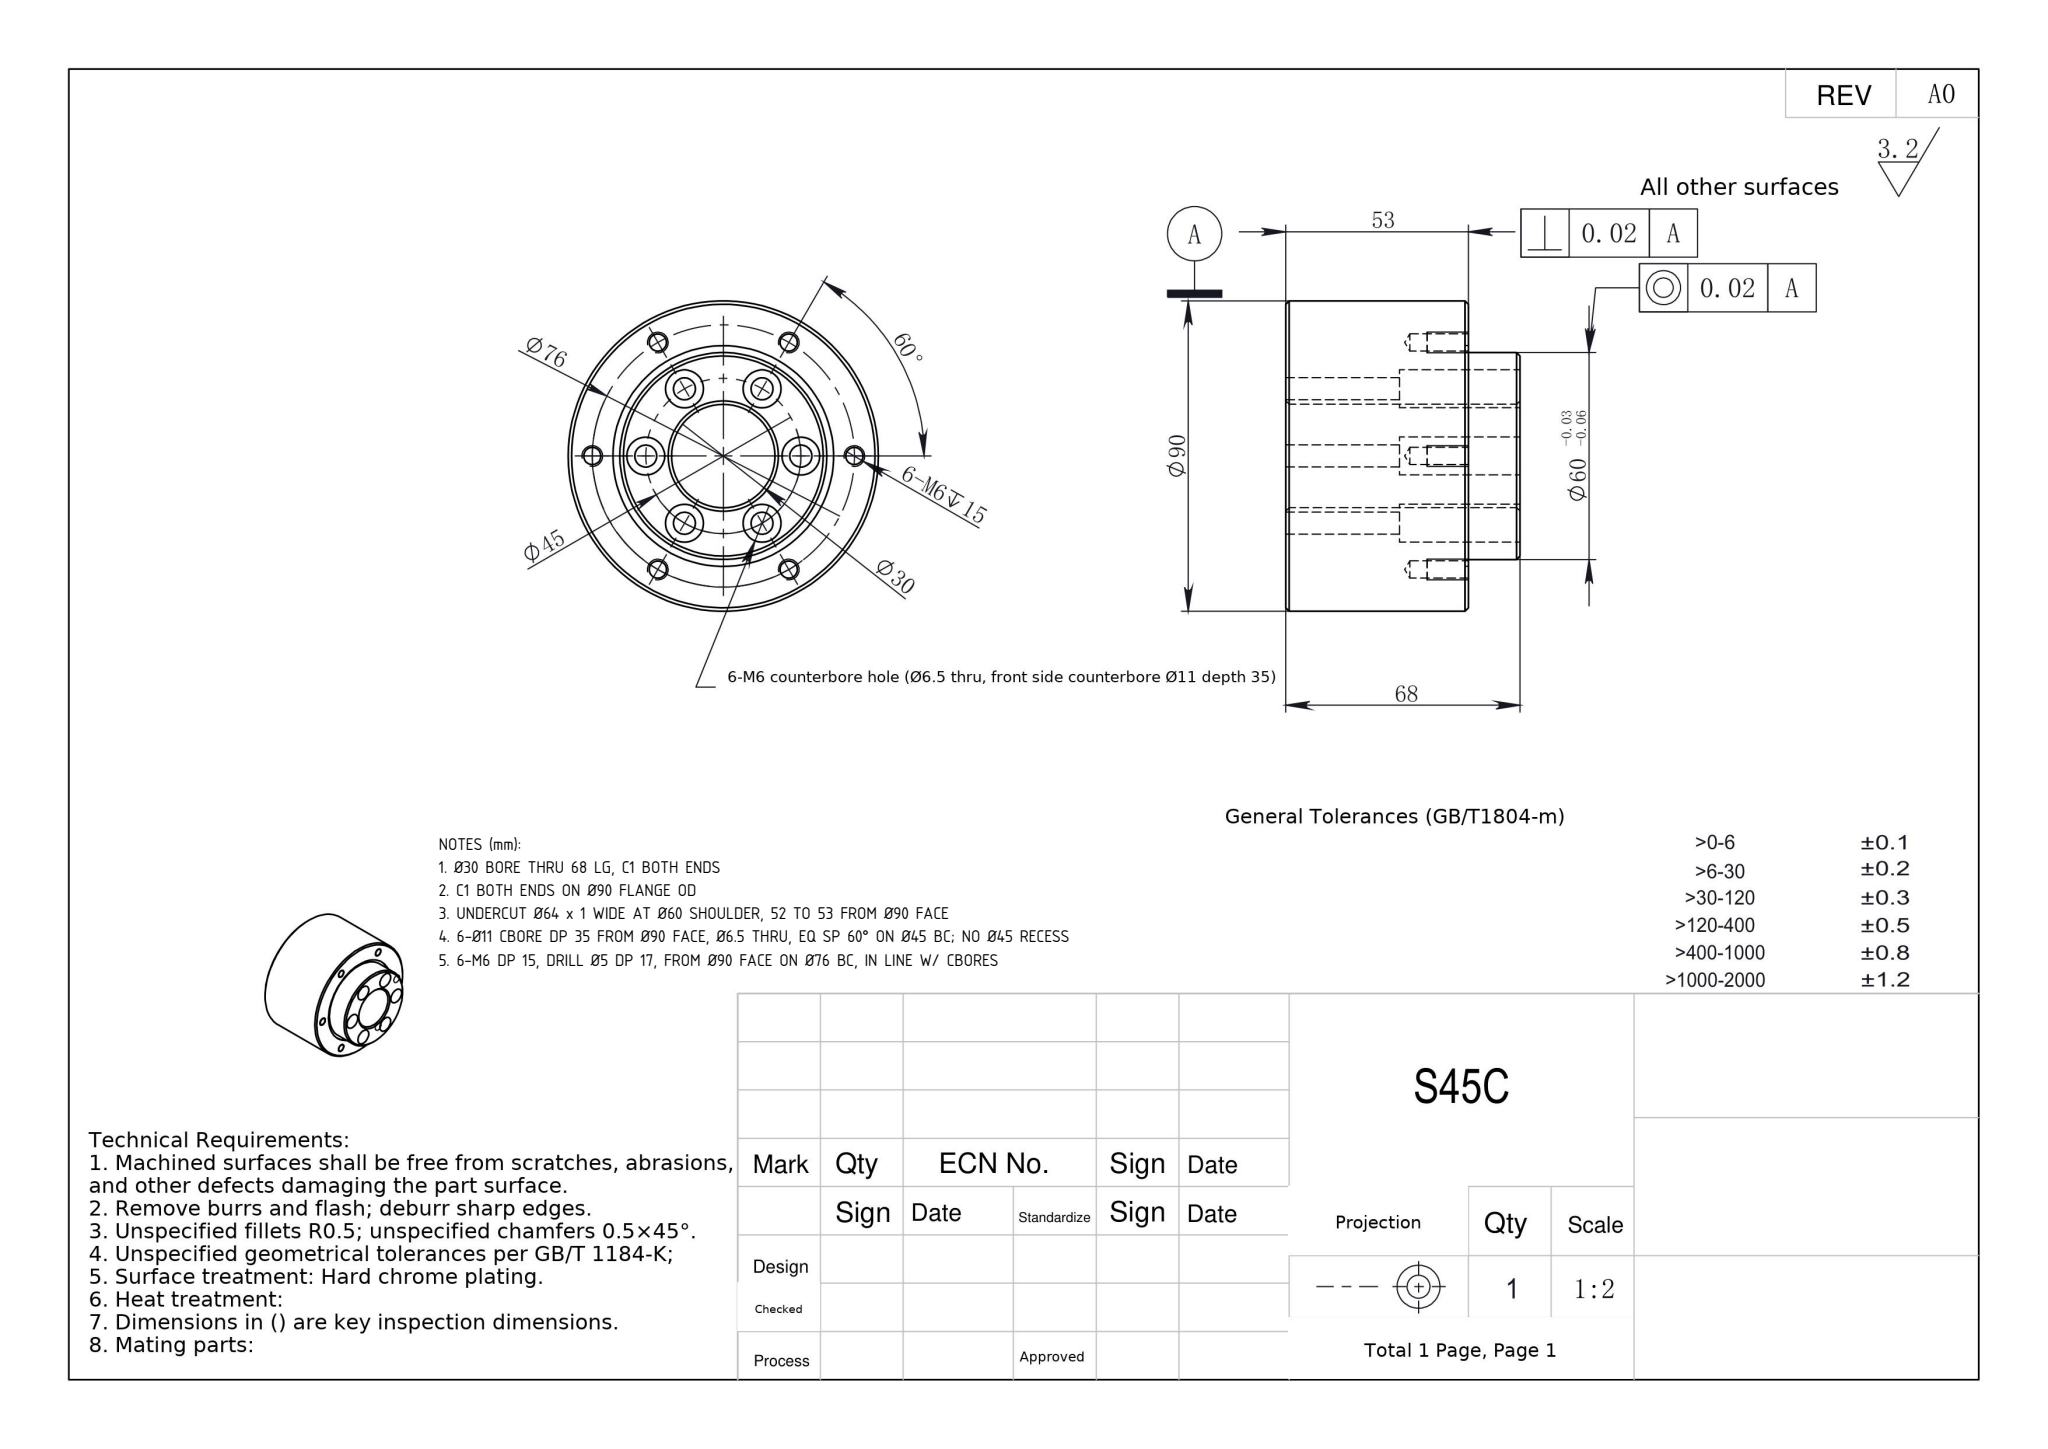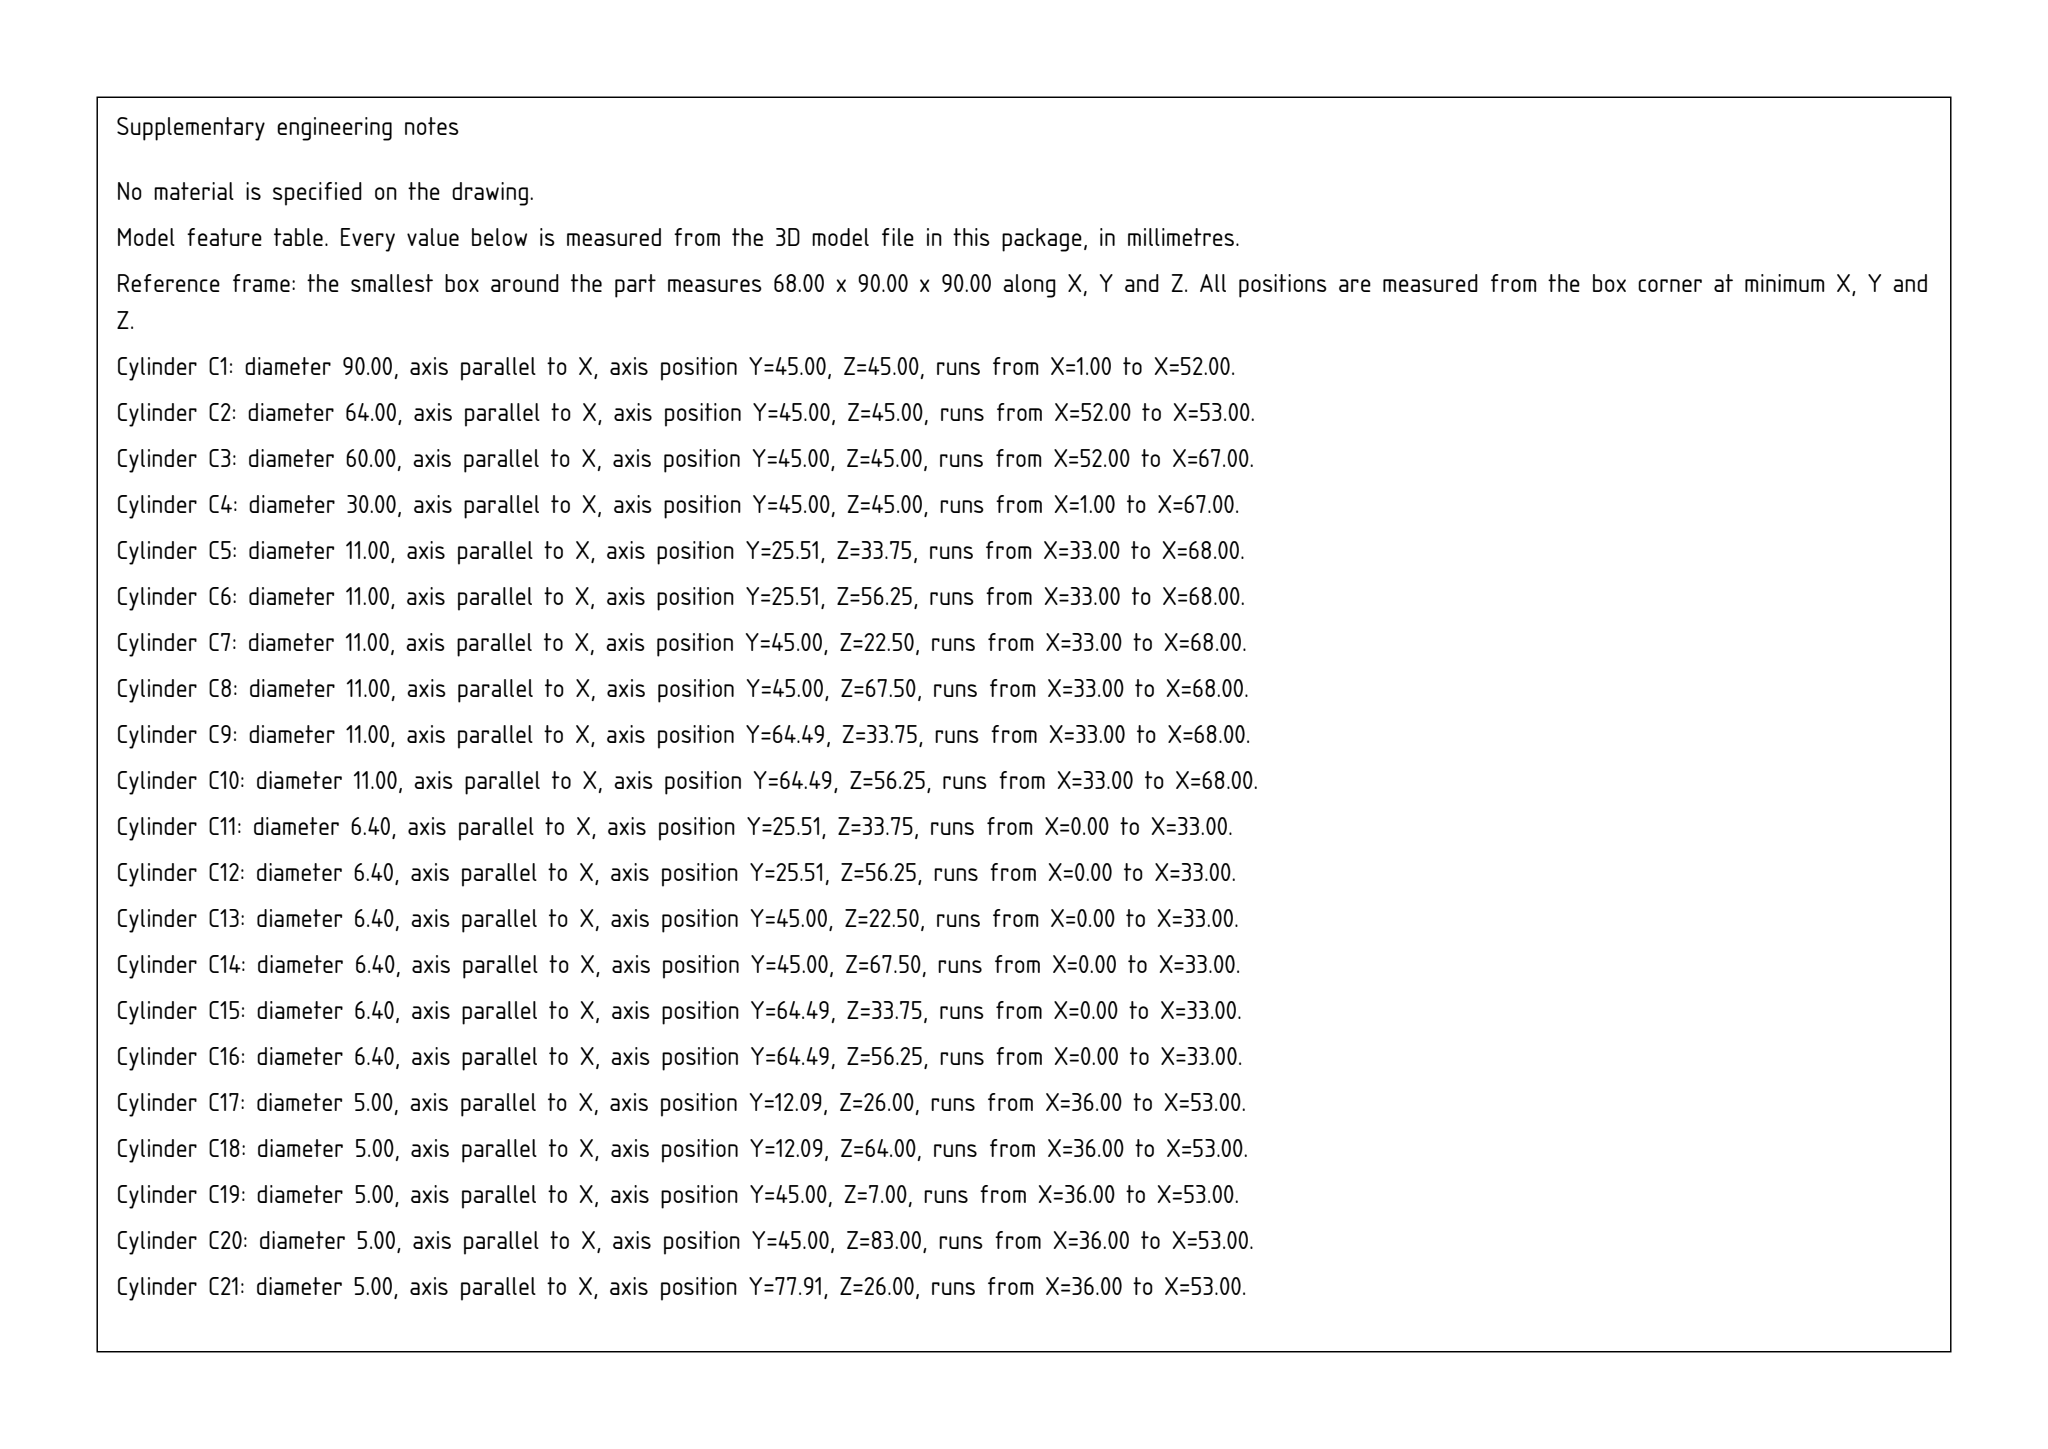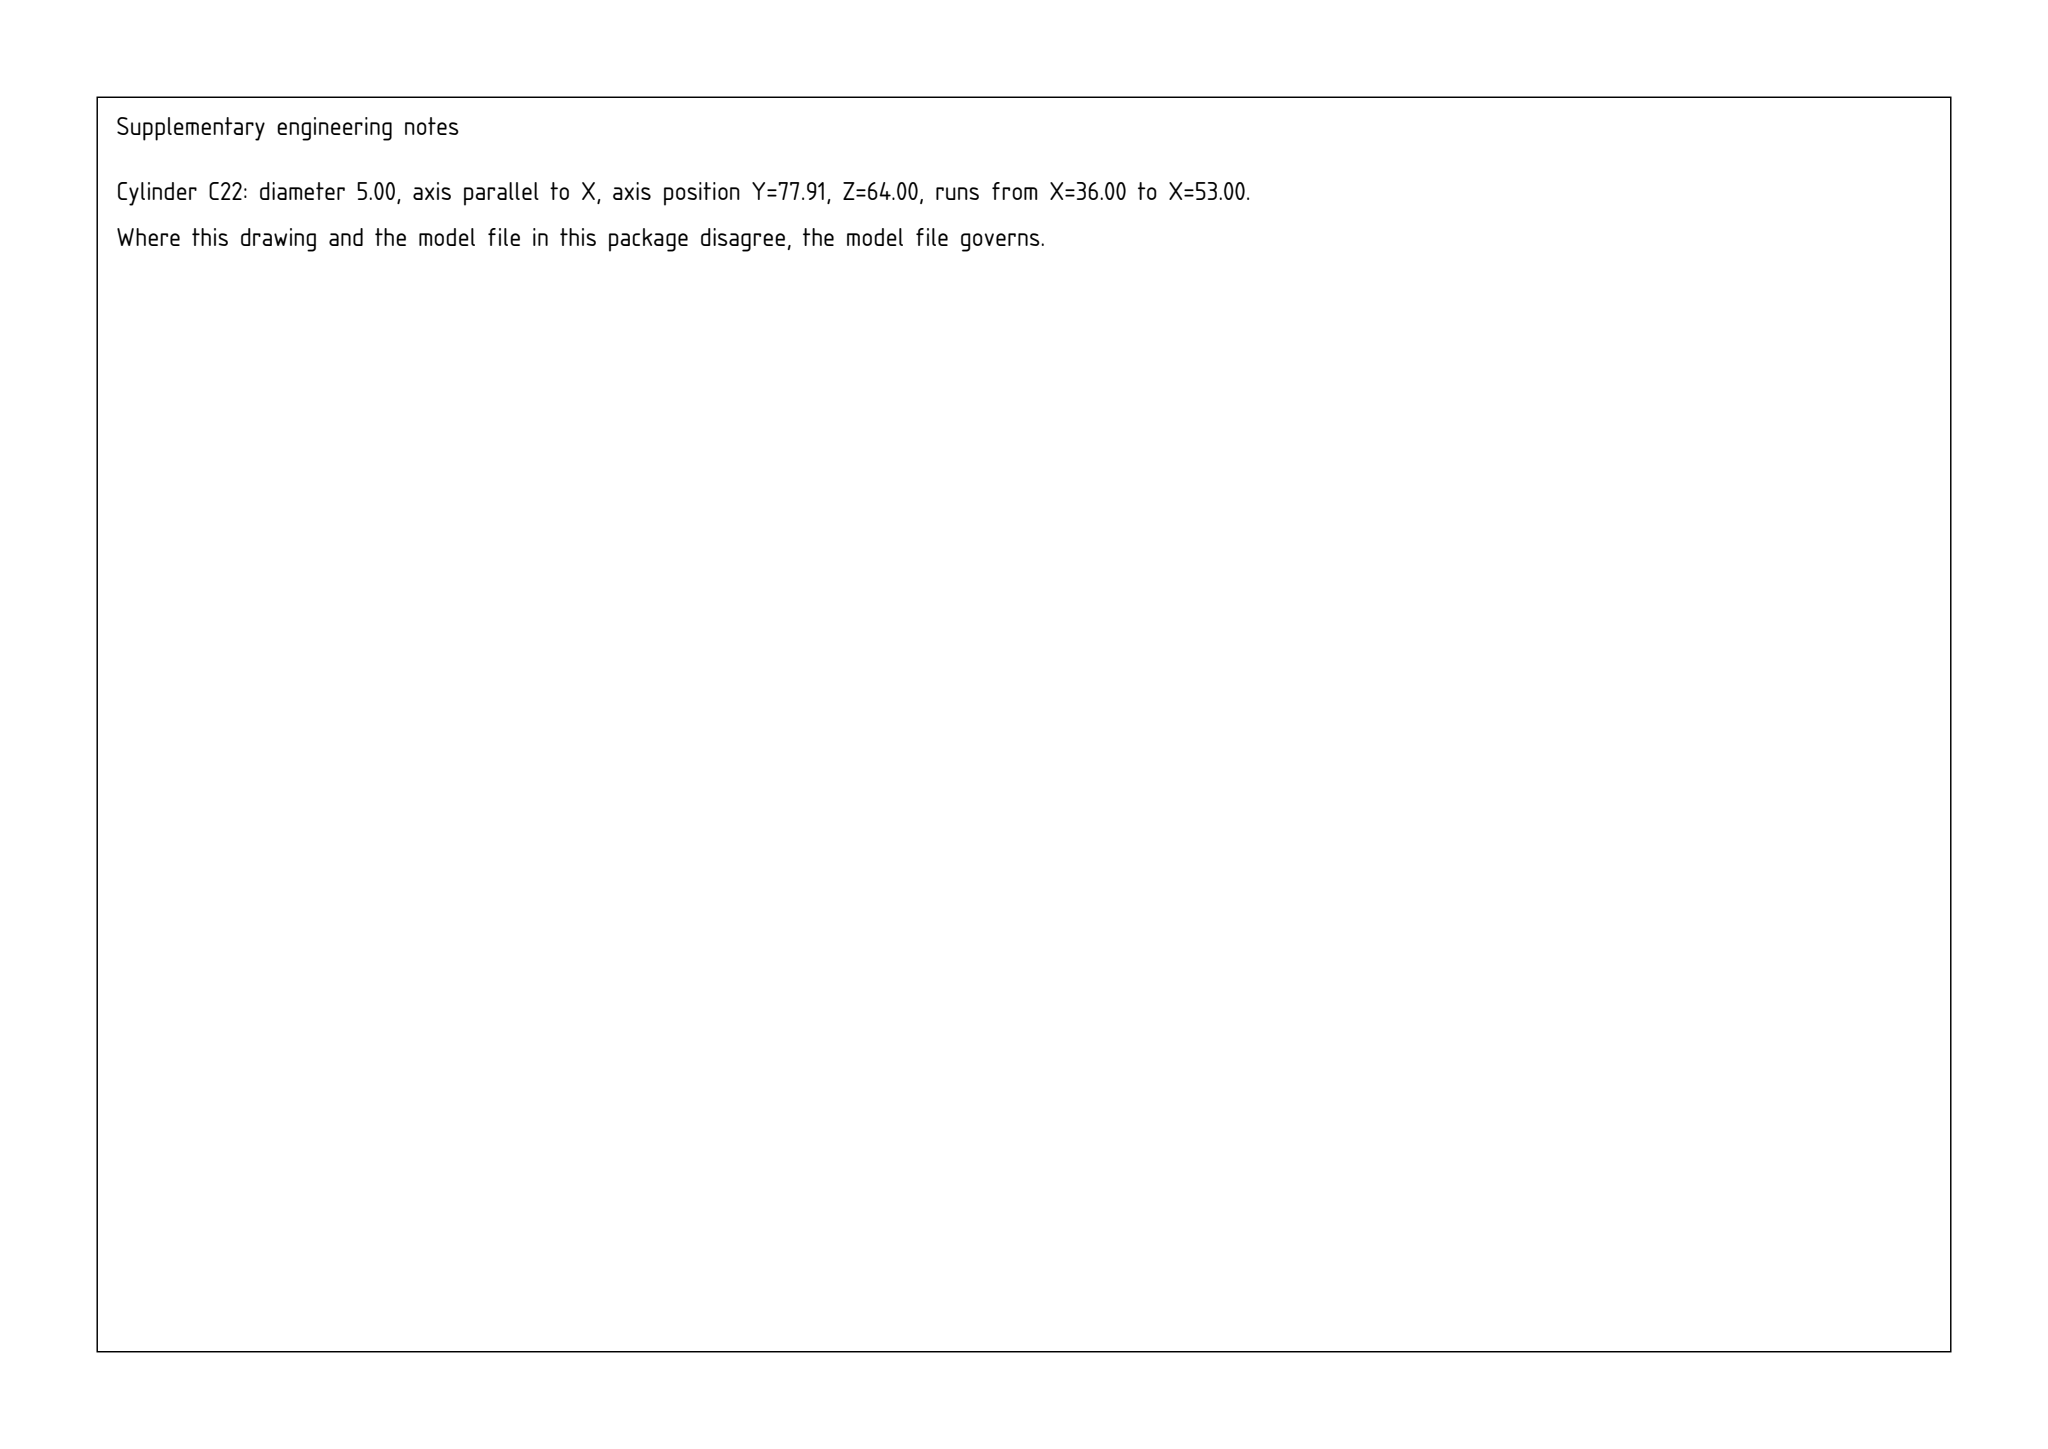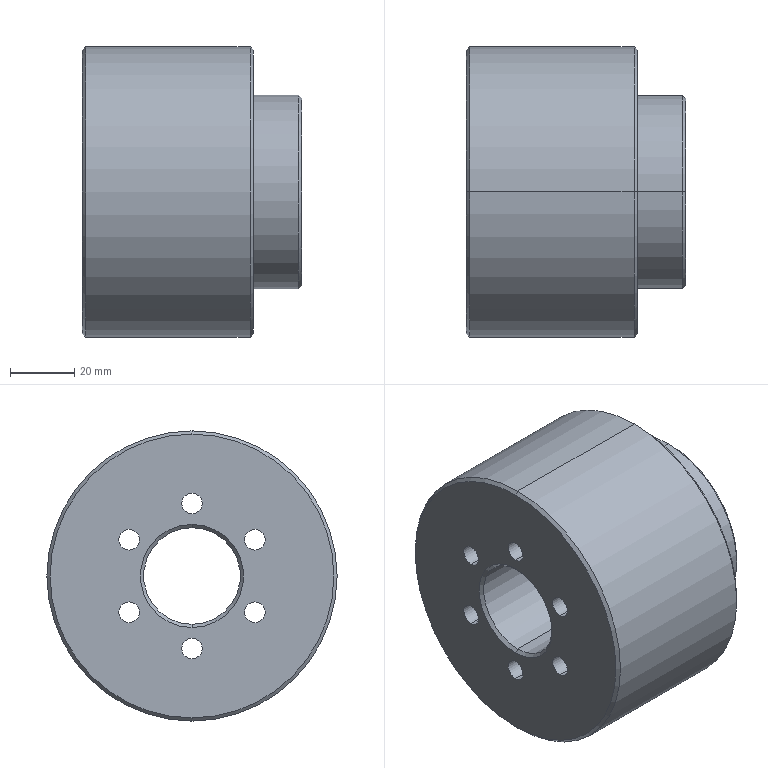Part | SolidWorks | mm | 1 solid | 76 faces | box 68 x 90 x 90 mm | volume 302268 mm3 | cylinder 44 | cone 22 | plane 10 | commonest cylinder face diameters 11 x12 6.4 x12 5 x12 60 x2 64 x2 90 x2 30 x2
Drawing notes:
Ø30 BORE THRU 68 LG, C1 BOTH ENDS | from the solid: Ø30 cyl L=66 on x axis + 90° cones ref Ø30/Ø32 each end = 68 total = bbox X
C1 BOTH ENDS ON Ø90 FLANGE OD | from the solid: 90° cones ref dia 90 and 88 at x=0-1 and x=52-53 => 1x45°
UNDERCUT Ø64 x 1 WIDE AT Ø60 SHOULDER, 52 TO 53 FROM Ø90 FACE | from the solid: Cyl Ø64 axis x L=1 spanning x=52 to 53; shoulder plane at x=53
6-Ø11 CBORE DP 35 FROM Ø90 FACE, Ø6.5 THRU, EQ SP 60° ON Ø45 BC; NO Ø45 RECESS | from the solid: Ø11 L=35 coaxial w/ Ø6.4 L=33 from x=0 face, at R22.5 about (45,45), 30/90/150/210/270/330°; no Ø45 cyl
6-M6 DP 15, DRILL Ø5 DP 17, FROM Ø90 FACE ON Ø76 BC, IN LINE W/ CBORES | from the solid: Ø5 cyls L=17 at R38 from x=0 face, 118° drill point, same angles as Ø11 cbores
build123d program:
from build123d import *

# Parameters (mm, degrees)
CIRPATTERN1_COUNT                                    = 6
HOLE_SIZE_ACCORDING_TO_THE_TYPE_OF_HEXAG_D           = 6.4
HOLE_SIZE_ACCORDING_TO_THE_TYPE_OF_HEXAG_CBORE_D     = 11
HOLE_SIZE_ACCORDING_TO_THE_TYPE_OF_HEXAG_CBORE_DEPTH = 35
CHAMFER1_SIZE                                        = 1
CHAMFER2_SIZE                                        = 1
CIRPATTERN2_COUNT                                    = 6


with BuildPart() as part:
    # Sketch1 → Revolve1 (revolve)
    with BuildSketch(Plane(origin=(0, 0, 0), x_dir=(1, 0, 0), z_dir=(0, 1, 0)), mode=Mode.PRIVATE) as revolve1_sk:
        Polygon((0, 15), (0, 45), (53, 45), (53, 32), (52, 32), (52, 30), (63, 30), (68, 30), (68, 15), align=None)
    revolve(revolve1_sk.sketch.rotate(Axis((0, 0, 0), (1, 0, 0)), 180), axis=Axis((0, 0, 0), (1, 0, 0)))

    # Sketch2 → M6 Tapped Hole1 (revolve, cut)
    with BuildSketch(Plane(origin=(53, 0, -38), x_dir=(0, 0, -1), z_dir=(0, 1, 0))):
        Polygon((0, 0), (0, 18.502), (2.5, 17), (2.5, 0), align=None)
    m6_tapped_hole1 = revolve(axis=Axis((59.35, 0, -38), (-1, 0, 0)), mode=Mode.SUBTRACT)

    # CirPattern1: M6 Tapped Hole1 ×6 about axis
    cirpattern1_axis = Axis((0, 0, 0), (1, 0, 0))
    for i in range(1, CIRPATTERN1_COUNT):
        add(m6_tapped_hole1.rotate(cirpattern1_axis, i * 360 / CIRPATTERN1_COUNT), mode=Mode.SUBTRACT)

    # Hole size according to the type of hexag (through all)
    with Locations(Plane(origin=(68, 0, 0), x_dir=(0, 0, -1), z_dir=(1, 0, 0))):
        with Locations((11.25, 19.486)):
            hole_size_according_to_the_type_of_hexag = CounterBoreHole(HOLE_SIZE_ACCORDING_TO_THE_TYPE_OF_HEXAG_D / 2, HOLE_SIZE_ACCORDING_TO_THE_TYPE_OF_HEXAG_CBORE_D / 2, HOLE_SIZE_ACCORDING_TO_THE_TYPE_OF_HEXAG_CBORE_DEPTH)

    # Chamfer1
    chamfer1_edges = [part.edges().sort_by_distance(p)[0] for p in [
        (0, 0, -15),
        (68, 0, -15),
    ]]
    chamfer(chamfer1_edges, length=CHAMFER1_SIZE)

    # Chamfer2
    chamfer2_edges = [part.edges().sort_by_distance(p)[0] for p in [
        (68, 0, -30),
        (53, 0, -45),
        (0, 0, -45),
    ]]
    chamfer(chamfer2_edges, length=CHAMFER2_SIZE)

    # CirPattern2: Hole size according to the type of hexag ×6 about axis
    cirpattern2_axis = Axis((0, 0, 0), (1, 0, 0))
    for i in range(1, CIRPATTERN2_COUNT):
        add(hole_size_according_to_the_type_of_hexag.rotate(cirpattern2_axis, i * 360 / CIRPATTERN2_COUNT), mode=Mode.SUBTRACT)


solid = part.part